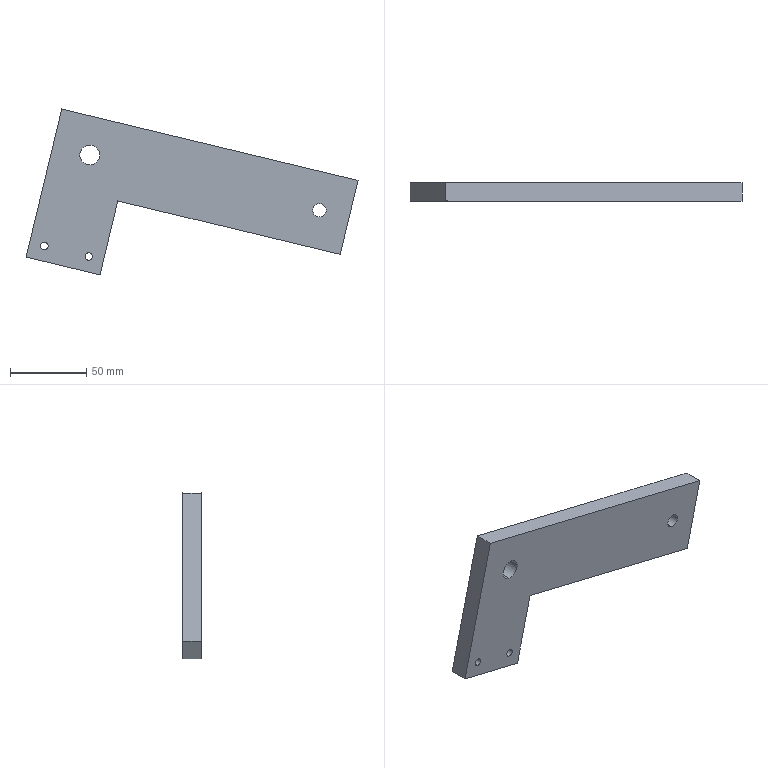Component | SolidWorks | SpringPullPlate-1 | 1 solid | 16 faces | box 217.86 x 12 x 108.93 mm | volume 147206 mm3 | cylinder 8 | plane 8 | commonest cylinder face diameters 5 x4 8.8 x2 13 x2
build123d program:
from build123d import *

# Parameters (mm, degrees)
SKETCH1_R                   = 6.5
EXTRUDE1_DEPTH              = 12
M10X1_25_TAPPED_HOLE1_D     = 8.8
M10X1_25_TAPPED_HOLE1_DEPTH = 26.25
M10X1_25_TAPPED_HOLE1_TIP   = 2.644
M6_TAPPED_HOLE1_D           = 5
M6_TAPPED_HOLE1_DEPTH       = 17
M6_TAPPED_HOLE1_TIP         = 1.502


with BuildPart() as part:
    # Sketch1 → Extrude1 (new body)
    with BuildSketch(Plane.XY):
        Polygon((-30.524, 33.502), (-30.524, -166.498), (69.476, -166.498), (69.476, -116.498), (19.476, -116.498), (19.476, 33.502), align=None)
        with Locations((-5.524, -141.498)):
            Circle(SKETCH1_R, mode=Mode.SUBTRACT)
    extrude(amount=EXTRUDE1_DEPTH)

    # M10x1.25 Tapped Hole1
    with Locations(Plane(origin=(-5.524, 13.502, 12), x_dir=(1, 0, 0), z_dir=(0, 0, 1))):
        with Locations((0, 0)):
            Hole(M10X1_25_TAPPED_HOLE1_D / 2, depth=M10X1_25_TAPPED_HOLE1_DEPTH)
            with Locations((0, 0, -(M10X1_25_TAPPED_HOLE1_DEPTH + M10X1_25_TAPPED_HOLE1_TIP / 2))):  # 118° drill point
                Cone(0, M10X1_25_TAPPED_HOLE1_D / 2, M10X1_25_TAPPED_HOLE1_TIP, mode=Mode.SUBTRACT)

    # M6 Tapped Hole1
    with Locations(Plane(origin=(59.476, -126.498, 12), x_dir=(1, 0, 0), z_dir=(0, 0, 1))):
        with Locations((0, 0), (0, -30)):
            Hole(M6_TAPPED_HOLE1_D / 2, depth=M6_TAPPED_HOLE1_DEPTH)
            with Locations((0, 0, -(M6_TAPPED_HOLE1_DEPTH + M6_TAPPED_HOLE1_TIP / 2))):  # 118° drill point
                Cone(0, M6_TAPPED_HOLE1_D / 2, M6_TAPPED_HOLE1_TIP, mode=Mode.SUBTRACT)


solid = part.part

# Placed as in the assembly
solid = solid.moved(Location((386.487, 406.983, -247.005), (90, 0, -103.543)))
STEP:
#1=CARTESIAN_POINT('',(9.849,16.023,-10.739));
#2=VERTEX_POINT('',#1);
#3=CARTESIAN_POINT('',(9.803,16.023,-10.931));
#4=VERTEX_POINT('',#3);
#5=CARTESIAN_POINT('',(9.826,16.023,-10.835));
#6=DIRECTION('',(-0.,-1.,0.));
#7=DIRECTION('',(-0.2342,0.,-0.9722));
#8=AXIS2_PLACEMENT_3D('',#5,#6,#7);
#9=CIRCLE('',#8,0.09843);
#10=EDGE_CURVE('',#2,#4,#9,.T.);
#11=ORIENTED_EDGE('',*,*,#10,.F.);
#12=CARTESIAN_POINT('',(9.849,15.551,-10.739));
#13=VERTEX_POINT('',#12);
#14=CARTESIAN_POINT('',(9.849,15.551,-10.739));
#15=DIRECTION('',(-0.,-1.,0.));
#16=VECTOR('',#15,39.37);
#17=LINE('',#14,#16);
#18=EDGE_CURVE('',#2,#13,#17,.T.);
#19=ORIENTED_EDGE('',*,*,#18,.T.);
#20=CARTESIAN_POINT('',(9.803,15.551,-10.931));
#21=VERTEX_POINT('',#20);
#22=CARTESIAN_POINT('',(9.826,15.551,-10.835));
#23=DIRECTION('',(-0.,-1.,0.));
#24=DIRECTION('',(-0.2342,0.,-0.9722));
#25=AXIS2_PLACEMENT_3D('',#22,#23,#24);
#26=CIRCLE('',#25,0.09843);
#27=EDGE_CURVE('',#13,#21,#26,.T.);
#28=ORIENTED_EDGE('',*,*,#27,.T.);
#29=CARTESIAN_POINT('',(9.803,15.551,-10.931));
#30=DIRECTION('',(-0.,-1.,0.));
#31=VECTOR('',#30,39.37);
#32=LINE('',#29,#31);
#33=EDGE_CURVE('',#4,#21,#32,.T.);
#34=ORIENTED_EDGE('',*,*,#33,.F.);
#35=EDGE_LOOP('',(#11,#19,#28,#34));
#36=FACE_OUTER_BOUND('',#35,.T.);
#37=CARTESIAN_POINT('',(9.826,15.551,-10.835));
#38=DIRECTION('',(-0.,-1.,0.));
#39=DIRECTION('',(-0.2342,0.,-0.9722));
#40=AXIS2_PLACEMENT_3D('',#37,#38,#39);
#41=CYLINDRICAL_SURFACE('',#40,0.09843);
#42=ADVANCED_FACE('',(#36),#41,.F.);
#43=CARTESIAN_POINT('',(8.701,16.023,-10.463));
#44=VERTEX_POINT('',#43);
#45=CARTESIAN_POINT('',(8.655,16.023,-10.654));
#46=VERTEX_POINT('',#45);
#47=CARTESIAN_POINT('',(8.678,16.023,-10.558));
#48=DIRECTION('',(-0.,-1.,0.));
#49=DIRECTION('',(-0.2342,0.,-0.9722));
#50=AXIS2_PLACEMENT_3D('',#47,#48,#49);
#51=CIRCLE('',#50,0.09843);
#52=EDGE_CURVE('',#44,#46,#51,.T.);
#53=ORIENTED_EDGE('',*,*,#52,.F.);
#54=CARTESIAN_POINT('',(8.701,15.551,-10.463));
#55=VERTEX_POINT('',#54);
#56=CARTESIAN_POINT('',(8.701,15.551,-10.463));
#57=DIRECTION('',(-0.,-1.,0.));
#58=VECTOR('',#57,39.37);
#59=LINE('',#56,#58);
#60=EDGE_CURVE('',#44,#55,#59,.T.);
#61=ORIENTED_EDGE('',*,*,#60,.T.);
#62=CARTESIAN_POINT('',(8.655,15.551,-10.654));
#63=VERTEX_POINT('',#62);
#64=CARTESIAN_POINT('',(8.678,15.551,-10.558));
#65=DIRECTION('',(-0.,-1.,0.));
#66=DIRECTION('',(-0.2342,0.,-0.9722));
#67=AXIS2_PLACEMENT_3D('',#64,#65,#66);
#68=CIRCLE('',#67,0.09843);
#69=EDGE_CURVE('',#55,#63,#68,.T.);
#70=ORIENTED_EDGE('',*,*,#69,.T.);
#71=CARTESIAN_POINT('',(8.655,15.551,-10.654));
#72=DIRECTION('',(-0.,-1.,0.));
#73=VECTOR('',#72,39.37);
#74=LINE('',#71,#73);
#75=EDGE_CURVE('',#46,#63,#74,.T.);
#76=ORIENTED_EDGE('',*,*,#75,.F.);
#77=EDGE_LOOP('',(#53,#61,#70,#76));
#78=FACE_OUTER_BOUND('',#77,.T.);
#79=CARTESIAN_POINT('',(8.678,15.551,-10.558));
#80=DIRECTION('',(-0.,-1.,0.));
#81=DIRECTION('',(-0.2342,0.,-0.9722));
#82=AXIS2_PLACEMENT_3D('',#79,#80,#81);
#83=CYLINDRICAL_SURFACE('',#82,0.09843);
#84=ADVANCED_FACE('',(#78),#83,.F.);
#85=CARTESIAN_POINT('',(15.824,16.023,-9.469));
#86=VERTEX_POINT('',#85);
#87=CARTESIAN_POINT('',(15.743,16.023,-9.806));
#88=VERTEX_POINT('',#87);
#89=CARTESIAN_POINT('',(15.784,16.023,-9.638));
#90=DIRECTION('',(-0.,-1.,0.));
#91=DIRECTION('',(-0.2342,0.,-0.9722));
#92=AXIS2_PLACEMENT_3D('',#89,#90,#91);
#93=CIRCLE('',#92,0.1732);
#94=EDGE_CURVE('',#86,#88,#93,.T.);
#95=ORIENTED_EDGE('',*,*,#94,.F.);
#96=CARTESIAN_POINT('',(15.824,15.551,-9.469));
#97=VERTEX_POINT('',#96);
#98=CARTESIAN_POINT('',(15.824,15.551,-9.469));
#99=DIRECTION('',(-0.,-1.,0.));
#100=VECTOR('',#99,39.37);
#101=LINE('',#98,#100);
#102=EDGE_CURVE('',#86,#97,#101,.T.);
#103=ORIENTED_EDGE('',*,*,#102,.T.);
#104=CARTESIAN_POINT('',(15.743,15.551,-9.806));
#105=VERTEX_POINT('',#104);
#106=CARTESIAN_POINT('',(15.784,15.551,-9.638));
#107=DIRECTION('',(-0.,-1.,0.));
#108=DIRECTION('',(-0.2342,0.,-0.9722));
#109=AXIS2_PLACEMENT_3D('',#106,#107,#108);
#110=CIRCLE('',#109,0.1732);
#111=EDGE_CURVE('',#97,#105,#110,.T.);
#112=ORIENTED_EDGE('',*,*,#111,.T.);
#113=CARTESIAN_POINT('',(15.743,15.551,-9.806));
#114=DIRECTION('',(-0.,-1.,0.));
#115=VECTOR('',#114,39.37);
#116=LINE('',#113,#115);
#117=EDGE_CURVE('',#88,#105,#116,.T.);
#118=ORIENTED_EDGE('',*,*,#117,.F.);
#119=EDGE_LOOP('',(#95,#103,#112,#118));
#120=FACE_OUTER_BOUND('',#119,.T.);
#121=CARTESIAN_POINT('',(15.784,15.551,-9.638));
#122=DIRECTION('',(-0.,-1.,0.));
#123=DIRECTION('',(-0.2342,0.,-0.9722));
#124=AXIS2_PLACEMENT_3D('',#121,#122,#123);
#125=CYLINDRICAL_SURFACE('',#124,0.1732);
#126=ADVANCED_FACE('',(#120),#125,.F.);
#127=CARTESIAN_POINT('',(9.911,15.551,-7.96));
#128=VERTEX_POINT('',#127);
#129=CARTESIAN_POINT('',(9.791,15.551,-8.457));
#130=VERTEX_POINT('',#129);
#131=CARTESIAN_POINT('',(9.851,15.551,-8.209));
#132=DIRECTION('',(-0.,-1.,0.));
#133=DIRECTION('',(-0.2342,0.,-0.9722));
#134=AXIS2_PLACEMENT_3D('',#131,#132,#133);
#135=CIRCLE('',#134,0.2559);
#136=EDGE_CURVE('',#128,#130,#135,.T.);
#137=ORIENTED_EDGE('',*,*,#136,.T.);
#138=CARTESIAN_POINT('',(9.791,16.023,-8.457));
#139=VERTEX_POINT('',#138);
#140=CARTESIAN_POINT('',(9.791,15.551,-8.457));
#141=DIRECTION('',(0.,1.,-0.));
#142=VECTOR('',#141,39.37);
#143=LINE('',#140,#142);
#144=EDGE_CURVE('',#130,#139,#143,.T.);
#145=ORIENTED_EDGE('',*,*,#144,.T.);
#146=CARTESIAN_POINT('',(9.911,16.023,-7.96));
#147=VERTEX_POINT('',#146);
#148=CARTESIAN_POINT('',(9.851,16.023,-8.209));
#149=DIRECTION('',(-0.,-1.,0.));
#150=DIRECTION('',(-0.2342,0.,-0.9722));
#151=AXIS2_PLACEMENT_3D('',#148,#149,#150);
#152=CIRCLE('',#151,0.2559);
#153=EDGE_CURVE('',#147,#139,#152,.T.);
#154=ORIENTED_EDGE('',*,*,#153,.F.);
#155=CARTESIAN_POINT('',(9.911,15.551,-7.96));
#156=DIRECTION('',(0.,1.,-0.));
#157=VECTOR('',#156,39.37);
#158=LINE('',#155,#157);
#159=EDGE_CURVE('',#128,#147,#158,.T.);
#160=ORIENTED_EDGE('',*,*,#159,.F.);
#161=EDGE_LOOP('',(#137,#145,#154,#160));
#162=FACE_OUTER_BOUND('',#161,.T.);
#163=CARTESIAN_POINT('',(9.851,15.551,-8.209));
#164=DIRECTION('',(0.,1.,-0.));
#165=DIRECTION('',(0.2342,0.,0.9722));
#166=AXIS2_PLACEMENT_3D('',#163,#164,#165);
#167=CYLINDRICAL_SURFACE('',#166,0.2559);
#168=ADVANCED_FACE('',(#162),#167,.F.);
#169=CARTESIAN_POINT('',(9.826,15.551,-10.835));
#170=DIRECTION('',(-0.,-1.,0.));
#171=DIRECTION('',(-0.2342,0.,-0.9722));
#172=AXIS2_PLACEMENT_3D('',#169,#170,#171);
#173=CIRCLE('',#172,0.09843);
#174=EDGE_CURVE('',#21,#13,#173,.T.);
#175=ORIENTED_EDGE('',*,*,#174,.F.);
#176=ORIENTED_EDGE('',*,*,#27,.F.);
#177=EDGE_LOOP('',(#175,#176));
#178=FACE_BOUND('',#177,.T.);
#179=CARTESIAN_POINT('',(8.678,15.551,-10.558));
#180=DIRECTION('',(-0.,-1.,0.));
#181=DIRECTION('',(-0.2342,0.,-0.9722));
#182=AXIS2_PLACEMENT_3D('',#179,#180,#181);
#183=CIRCLE('',#182,0.09843);
#184=EDGE_CURVE('',#63,#55,#183,.T.);
#185=ORIENTED_EDGE('',*,*,#184,.F.);
#186=ORIENTED_EDGE('',*,*,#69,.F.);
#187=EDGE_LOOP('',(#185,#186));
#188=FACE_BOUND('',#187,.T.);
#189=CARTESIAN_POINT('',(15.784,15.551,-9.638));
#190=DIRECTION('',(-0.,-1.,0.));
#191=DIRECTION('',(-0.2342,0.,-0.9722));
#192=AXIS2_PLACEMENT_3D('',#189,#190,#191);
#193=CIRCLE('',#192,0.1732);
#194=EDGE_CURVE('',#105,#97,#193,.T.);
#195=ORIENTED_EDGE('',*,*,#194,.F.);
#196=ORIENTED_EDGE('',*,*,#111,.F.);
#197=EDGE_LOOP('',(#195,#196));
#198=FACE_BOUND('',#197,.T.);
#199=CARTESIAN_POINT('',(9.125,15.551,-7.021));
#200=VERTEX_POINT('',#199);
#201=CARTESIAN_POINT('',(8.203,15.551,-10.849));
#202=VERTEX_POINT('',#201);
#203=CARTESIAN_POINT('',(9.125,15.551,-7.021));
#204=DIRECTION('',(-0.2342,-0.,-0.9722));
#205=VECTOR('',#204,39.37);
#206=LINE('',#203,#205);
#207=EDGE_CURVE('',#200,#202,#206,.T.);
#208=ORIENTED_EDGE('',*,*,#207,.T.);
#209=CARTESIAN_POINT('',(10.116,15.551,-11.31));
#210=VERTEX_POINT('',#209);
#211=CARTESIAN_POINT('',(8.203,15.551,-10.849));
#212=DIRECTION('',(0.9722,-0.,-0.2342));
#213=VECTOR('',#212,39.37);
#214=LINE('',#211,#213);
#215=EDGE_CURVE('',#202,#210,#214,.T.);
#216=ORIENTED_EDGE('',*,*,#215,.T.);
#217=CARTESIAN_POINT('',(10.577,15.551,-9.396));
#218=VERTEX_POINT('',#217);
#219=CARTESIAN_POINT('',(10.116,15.551,-11.31));
#220=DIRECTION('',(0.2342,0.,0.9722));
#221=VECTOR('',#220,39.37);
#222=LINE('',#219,#221);
#223=EDGE_CURVE('',#210,#218,#222,.T.);
#224=ORIENTED_EDGE('',*,*,#223,.T.);
#225=CARTESIAN_POINT('',(16.319,15.551,-10.779));
#226=VERTEX_POINT('',#225);
#227=CARTESIAN_POINT('',(10.577,15.551,-9.396));
#228=DIRECTION('',(0.9722,-0.,-0.2342));
#229=VECTOR('',#228,39.37);
#230=LINE('',#227,#229);
#231=EDGE_CURVE('',#218,#226,#230,.T.);
#232=ORIENTED_EDGE('',*,*,#231,.T.);
#233=CARTESIAN_POINT('',(16.78,15.551,-8.865));
#234=VERTEX_POINT('',#233);
#235=CARTESIAN_POINT('',(16.319,15.551,-10.779));
#236=DIRECTION('',(0.2342,0.,0.9722));
#237=VECTOR('',#236,39.37);
#238=LINE('',#235,#237);
#239=EDGE_CURVE('',#226,#234,#238,.T.);
#240=ORIENTED_EDGE('',*,*,#239,.T.);
#241=CARTESIAN_POINT('',(16.78,15.551,-8.865));
#242=DIRECTION('',(-0.9722,0.,0.2342));
#243=VECTOR('',#242,39.37);
#244=LINE('',#241,#243);
#245=EDGE_CURVE('',#234,#200,#244,.T.);
#246=ORIENTED_EDGE('',*,*,#245,.T.);
#247=EDGE_LOOP('',(#208,#216,#224,#232,#240,#246));
#248=FACE_OUTER_BOUND('',#247,.T.);
#249=ORIENTED_EDGE('',*,*,#136,.F.);
#250=CARTESIAN_POINT('',(9.851,15.551,-8.209));
#251=DIRECTION('',(-0.,-1.,0.));
#252=DIRECTION('',(-0.2342,0.,-0.9722));
#253=AXIS2_PLACEMENT_3D('',#250,#251,#252);
#254=CIRCLE('',#253,0.2559);
#255=EDGE_CURVE('',#130,#128,#254,.T.);
#256=ORIENTED_EDGE('',*,*,#255,.F.);
#257=EDGE_LOOP('',(#249,#256));
#258=FACE_BOUND('',#257,.T.);
#259=CARTESIAN_POINT('',(8.203,15.551,-10.849));
#260=DIRECTION('',(-0.,-1.,0.));
#261=DIRECTION('',(-0.2342,-0.,-0.9722));
#262=AXIS2_PLACEMENT_3D('',#259,#260,#261);
#263=PLANE('',#262);
#264=ADVANCED_FACE('',(#178,#188,#198,#248,#258),#263,.T.);
#265=CARTESIAN_POINT('',(9.826,16.023,-10.835));
#266=DIRECTION('',(-0.,-1.,0.));
#267=DIRECTION('',(-0.2342,0.,-0.9722));
#268=AXIS2_PLACEMENT_3D('',#265,#266,#267);
#269=CIRCLE('',#268,0.09843);
#270=EDGE_CURVE('',#4,#2,#269,.T.);
#271=ORIENTED_EDGE('',*,*,#270,.T.);
#272=ORIENTED_EDGE('',*,*,#10,.T.);
#273=EDGE_LOOP('',(#271,#272));
#274=FACE_BOUND('',#273,.T.);
#275=CARTESIAN_POINT('',(8.678,16.023,-10.558));
#276=DIRECTION('',(-0.,-1.,0.));
#277=DIRECTION('',(-0.2342,0.,-0.9722));
#278=AXIS2_PLACEMENT_3D('',#275,#276,#277);
#279=CIRCLE('',#278,0.09843);
#280=EDGE_CURVE('',#46,#44,#279,.T.);
#281=ORIENTED_EDGE('',*,*,#280,.T.);
#282=ORIENTED_EDGE('',*,*,#52,.T.);
#283=EDGE_LOOP('',(#281,#282));
#284=FACE_BOUND('',#283,.T.);
#285=CARTESIAN_POINT('',(15.784,16.023,-9.638));
#286=DIRECTION('',(-0.,-1.,0.));
#287=DIRECTION('',(-0.2342,0.,-0.9722));
#288=AXIS2_PLACEMENT_3D('',#285,#286,#287);
#289=CIRCLE('',#288,0.1732);
#290=EDGE_CURVE('',#88,#86,#289,.T.);
#291=ORIENTED_EDGE('',*,*,#290,.T.);
#292=ORIENTED_EDGE('',*,*,#94,.T.);
#293=EDGE_LOOP('',(#291,#292));
#294=FACE_BOUND('',#293,.T.);
#295=CARTESIAN_POINT('',(9.125,16.023,-7.021));
#296=VERTEX_POINT('',#295);
#297=CARTESIAN_POINT('',(8.203,16.023,-10.849));
#298=VERTEX_POINT('',#297);
#299=CARTESIAN_POINT('',(9.125,16.023,-7.021));
#300=DIRECTION('',(-0.2342,-0.,-0.9722));
#301=VECTOR('',#300,39.37);
#302=LINE('',#299,#301);
#303=EDGE_CURVE('',#296,#298,#302,.T.);
#304=ORIENTED_EDGE('',*,*,#303,.F.);
#305=CARTESIAN_POINT('',(16.78,16.023,-8.865));
#306=VERTEX_POINT('',#305);
#307=CARTESIAN_POINT('',(16.78,16.023,-8.865));
#308=DIRECTION('',(-0.9722,0.,0.2342));
#309=VECTOR('',#308,39.37);
#310=LINE('',#307,#309);
#311=EDGE_CURVE('',#306,#296,#310,.T.);
#312=ORIENTED_EDGE('',*,*,#311,.F.);
#313=CARTESIAN_POINT('',(16.319,16.023,-10.779));
#314=VERTEX_POINT('',#313);
#315=CARTESIAN_POINT('',(16.319,16.023,-10.779));
#316=DIRECTION('',(0.2342,0.,0.9722));
#317=VECTOR('',#316,39.37);
#318=LINE('',#315,#317);
#319=EDGE_CURVE('',#314,#306,#318,.T.);
#320=ORIENTED_EDGE('',*,*,#319,.F.);
#321=CARTESIAN_POINT('',(10.577,16.023,-9.396));
#322=VERTEX_POINT('',#321);
#323=CARTESIAN_POINT('',(10.577,16.023,-9.396));
#324=DIRECTION('',(0.9722,-0.,-0.2342));
#325=VECTOR('',#324,39.37);
#326=LINE('',#323,#325);
#327=EDGE_CURVE('',#322,#314,#326,.T.);
#328=ORIENTED_EDGE('',*,*,#327,.F.);
#329=CARTESIAN_POINT('',(10.116,16.023,-11.31));
#330=VERTEX_POINT('',#329);
#331=CARTESIAN_POINT('',(10.116,16.023,-11.31));
#332=DIRECTION('',(0.2342,0.,0.9722));
#333=VECTOR('',#332,39.37);
#334=LINE('',#331,#333);
#335=EDGE_CURVE('',#330,#322,#334,.T.);
#336=ORIENTED_EDGE('',*,*,#335,.F.);
#337=CARTESIAN_POINT('',(8.203,16.023,-10.849));
#338=DIRECTION('',(0.9722,-0.,-0.2342));
#339=VECTOR('',#338,39.37);
#340=LINE('',#337,#339);
#341=EDGE_CURVE('',#298,#330,#340,.T.);
#342=ORIENTED_EDGE('',*,*,#341,.F.);
#343=EDGE_LOOP('',(#304,#312,#320,#328,#336,#342));
#344=FACE_OUTER_BOUND('',#343,.T.);
#345=ORIENTED_EDGE('',*,*,#153,.T.);
#346=CARTESIAN_POINT('',(9.851,16.023,-8.209));
#347=DIRECTION('',(-0.,-1.,0.));
#348=DIRECTION('',(-0.2342,0.,-0.9722));
#349=AXIS2_PLACEMENT_3D('',#346,#347,#348);
#350=CIRCLE('',#349,0.2559);
#351=EDGE_CURVE('',#139,#147,#350,.T.);
#352=ORIENTED_EDGE('',*,*,#351,.T.);
#353=EDGE_LOOP('',(#345,#352));
#354=FACE_BOUND('',#353,.T.);
#355=CARTESIAN_POINT('',(8.203,16.023,-10.849));
#356=DIRECTION('',(-0.,-1.,0.));
#357=DIRECTION('',(-0.2342,-0.,-0.9722));
#358=AXIS2_PLACEMENT_3D('',#355,#356,#357);
#359=PLANE('',#358);
#360=ADVANCED_FACE('',(#274,#284,#294,#344,#354),#359,.F.);
#361=ORIENTED_EDGE('',*,*,#303,.T.);
#362=CARTESIAN_POINT('',(8.203,15.551,-10.849));
#363=DIRECTION('',(0.,1.,-0.));
#364=VECTOR('',#363,39.37);
#365=LINE('',#362,#364);
#366=EDGE_CURVE('',#202,#298,#365,.T.);
#367=ORIENTED_EDGE('',*,*,#366,.F.);
#368=ORIENTED_EDGE('',*,*,#207,.F.);
#369=CARTESIAN_POINT('',(9.125,15.551,-7.021));
#370=DIRECTION('',(0.,1.,-0.));
#371=VECTOR('',#370,39.37);
#372=LINE('',#369,#371);
#373=EDGE_CURVE('',#200,#296,#372,.T.);
#374=ORIENTED_EDGE('',*,*,#373,.T.);
#375=EDGE_LOOP('',(#361,#367,#368,#374));
#376=FACE_OUTER_BOUND('',#375,.T.);
#377=CARTESIAN_POINT('',(9.125,15.551,-7.021));
#378=DIRECTION('',(0.9722,-0.,-0.2342));
#379=DIRECTION('',(-0.,-1.,0.));
#380=AXIS2_PLACEMENT_3D('',#377,#378,#379);
#381=PLANE('',#380);
#382=ADVANCED_FACE('',(#376),#381,.F.);
#383=ORIENTED_EDGE('',*,*,#341,.T.);
#384=CARTESIAN_POINT('',(10.116,15.551,-11.31));
#385=DIRECTION('',(0.,1.,-0.));
#386=VECTOR('',#385,39.37);
#387=LINE('',#384,#386);
#388=EDGE_CURVE('',#210,#330,#387,.T.);
#389=ORIENTED_EDGE('',*,*,#388,.F.);
#390=ORIENTED_EDGE('',*,*,#215,.F.);
#391=ORIENTED_EDGE('',*,*,#366,.T.);
#392=EDGE_LOOP('',(#383,#389,#390,#391));
#393=FACE_OUTER_BOUND('',#392,.T.);
#394=CARTESIAN_POINT('',(8.203,15.551,-10.849));
#395=DIRECTION('',(0.2342,0.,0.9722));
#396=DIRECTION('',(-0.,-1.,0.));
#397=AXIS2_PLACEMENT_3D('',#394,#395,#396);
#398=PLANE('',#397);
#399=ADVANCED_FACE('',(#393),#398,.F.);
#400=ORIENTED_EDGE('',*,*,#335,.T.);
#401=CARTESIAN_POINT('',(10.577,15.551,-9.396));
#402=DIRECTION('',(0.,1.,-0.));
#403=VECTOR('',#402,39.37);
#404=LINE('',#401,#403);
#405=EDGE_CURVE('',#218,#322,#404,.T.);
#406=ORIENTED_EDGE('',*,*,#405,.F.);
#407=ORIENTED_EDGE('',*,*,#223,.F.);
#408=ORIENTED_EDGE('',*,*,#388,.T.);
#409=EDGE_LOOP('',(#400,#406,#407,#408));
#410=FACE_OUTER_BOUND('',#409,.T.);
#411=CARTESIAN_POINT('',(10.116,15.551,-11.31));
#412=DIRECTION('',(-0.9722,0.,0.2342));
#413=DIRECTION('',(-0.2342,-0.,-0.9722));
#414=AXIS2_PLACEMENT_3D('',#411,#412,#413);
#415=PLANE('',#414);
#416=ADVANCED_FACE('',(#410),#415,.F.);
#417=ORIENTED_EDGE('',*,*,#327,.T.);
#418=CARTESIAN_POINT('',(16.319,15.551,-10.779));
#419=DIRECTION('',(0.,1.,-0.));
#420=VECTOR('',#419,39.37);
#421=LINE('',#418,#420);
#422=EDGE_CURVE('',#226,#314,#421,.T.);
#423=ORIENTED_EDGE('',*,*,#422,.F.);
#424=ORIENTED_EDGE('',*,*,#231,.F.);
#425=ORIENTED_EDGE('',*,*,#405,.T.);
#426=EDGE_LOOP('',(#417,#423,#424,#425));
#427=FACE_OUTER_BOUND('',#426,.T.);
#428=CARTESIAN_POINT('',(10.577,15.551,-9.396));
#429=DIRECTION('',(0.2342,0.,0.9722));
#430=DIRECTION('',(-0.,-1.,0.));
#431=AXIS2_PLACEMENT_3D('',#428,#429,#430);
#432=PLANE('',#431);
#433=ADVANCED_FACE('',(#427),#432,.F.);
#434=ORIENTED_EDGE('',*,*,#319,.T.);
#435=CARTESIAN_POINT('',(16.78,15.551,-8.865));
#436=DIRECTION('',(0.,1.,-0.));
#437=VECTOR('',#436,39.37);
#438=LINE('',#435,#437);
#439=EDGE_CURVE('',#234,#306,#438,.T.);
#440=ORIENTED_EDGE('',*,*,#439,.F.);
#441=ORIENTED_EDGE('',*,*,#239,.F.);
#442=ORIENTED_EDGE('',*,*,#422,.T.);
#443=EDGE_LOOP('',(#434,#440,#441,#442));
#444=FACE_OUTER_BOUND('',#443,.T.);
#445=CARTESIAN_POINT('',(16.319,15.551,-10.779));
#446=DIRECTION('',(-0.9722,0.,0.2342));
#447=DIRECTION('',(-0.2342,-0.,-0.9722));
#448=AXIS2_PLACEMENT_3D('',#445,#446,#447);
#449=PLANE('',#448);
#450=ADVANCED_FACE('',(#444),#449,.F.);
#451=ORIENTED_EDGE('',*,*,#311,.T.);
#452=ORIENTED_EDGE('',*,*,#373,.F.);
#453=ORIENTED_EDGE('',*,*,#245,.F.);
#454=ORIENTED_EDGE('',*,*,#439,.T.);
#455=EDGE_LOOP('',(#451,#452,#453,#454));
#456=FACE_OUTER_BOUND('',#455,.T.);
#457=CARTESIAN_POINT('',(16.78,15.551,-8.865));
#458=DIRECTION('',(-0.2342,-0.,-0.9722));
#459=DIRECTION('',(0.9722,-0.,-0.2342));
#460=AXIS2_PLACEMENT_3D('',#457,#458,#459);
#461=PLANE('',#460);
#462=ADVANCED_FACE('',(#456),#461,.F.);
#463=ORIENTED_EDGE('',*,*,#144,.F.);
#464=ORIENTED_EDGE('',*,*,#255,.T.);
#465=ORIENTED_EDGE('',*,*,#159,.T.);
#466=ORIENTED_EDGE('',*,*,#351,.F.);
#467=EDGE_LOOP('',(#463,#464,#465,#466));
#468=FACE_OUTER_BOUND('',#467,.T.);
#469=CARTESIAN_POINT('',(9.851,15.551,-8.209));
#470=DIRECTION('',(0.,1.,-0.));
#471=DIRECTION('',(0.2342,0.,0.9722));
#472=AXIS2_PLACEMENT_3D('',#469,#470,#471);
#473=CYLINDRICAL_SURFACE('',#472,0.2559);
#474=ADVANCED_FACE('',(#468),#473,.F.);
#475=ORIENTED_EDGE('',*,*,#102,.F.);
#476=ORIENTED_EDGE('',*,*,#290,.F.);
#477=ORIENTED_EDGE('',*,*,#117,.T.);
#478=ORIENTED_EDGE('',*,*,#194,.T.);
#479=EDGE_LOOP('',(#475,#476,#477,#478));
#480=FACE_OUTER_BOUND('',#479,.T.);
#481=CARTESIAN_POINT('',(15.784,15.551,-9.638));
#482=DIRECTION('',(-0.,-1.,0.));
#483=DIRECTION('',(-0.2342,0.,-0.9722));
#484=AXIS2_PLACEMENT_3D('',#481,#482,#483);
#485=CYLINDRICAL_SURFACE('',#484,0.1732);
#486=ADVANCED_FACE('',(#480),#485,.F.);
#487=ORIENTED_EDGE('',*,*,#60,.F.);
#488=ORIENTED_EDGE('',*,*,#280,.F.);
#489=ORIENTED_EDGE('',*,*,#75,.T.);
#490=ORIENTED_EDGE('',*,*,#184,.T.);
#491=EDGE_LOOP('',(#487,#488,#489,#490));
#492=FACE_OUTER_BOUND('',#491,.T.);
#493=CARTESIAN_POINT('',(8.678,15.551,-10.558));
#494=DIRECTION('',(-0.,-1.,0.));
#495=DIRECTION('',(-0.2342,0.,-0.9722));
#496=AXIS2_PLACEMENT_3D('',#493,#494,#495);
#497=CYLINDRICAL_SURFACE('',#496,0.09843);
#498=ADVANCED_FACE('',(#492),#497,.F.);
#499=ORIENTED_EDGE('',*,*,#18,.F.);
#500=ORIENTED_EDGE('',*,*,#270,.F.);
#501=ORIENTED_EDGE('',*,*,#33,.T.);
#502=ORIENTED_EDGE('',*,*,#174,.T.);
#503=EDGE_LOOP('',(#499,#500,#501,#502));
#504=FACE_OUTER_BOUND('',#503,.T.);
#505=CARTESIAN_POINT('',(9.826,15.551,-10.835));
#506=DIRECTION('',(-0.,-1.,0.));
#507=DIRECTION('',(-0.2342,0.,-0.9722));
#508=AXIS2_PLACEMENT_3D('',#505,#506,#507);
#509=CYLINDRICAL_SURFACE('',#508,0.09843);
#510=ADVANCED_FACE('',(#504),#509,.F.);
#511=CLOSED_SHELL('',(#42,#84,#126,#168,#264,#360,#382,#399,#416,#433,#450,#462,#474,#486,#498,#510));
#512=MANIFOLD_SOLID_BREP('',#511);
#513=CARTESIAN_POINT('',(0.,0.,0.));
#514=DIRECTION('',(0.,0.,1.));
#515=DIRECTION('',(1.,0.,0.));
#516=AXIS2_PLACEMENT_3D('',#513,#514,#515);
#517=(LENGTH_UNIT()NAMED_UNIT(*)SI_UNIT($,.METRE.));
#518=LENGTH_MEASURE_WITH_UNIT(LENGTH_MEASURE(0.0254),#517);
#519=DIMENSIONAL_EXPONENTS(1.,0.,0.,0.,0.,0.,0.);
#520=(CONVERSION_BASED_UNIT('',#518)LENGTH_UNIT()NAMED_UNIT(#519));
#521=UNCERTAINTY_MEASURE_WITH_UNIT(LENGTH_MEASURE(0.00001),#520,'','');
#522=(NAMED_UNIT(*)PLANE_ANGLE_UNIT()SI_UNIT($,.RADIAN.));
#523=(NAMED_UNIT(*)SI_UNIT($,.STERADIAN.)SOLID_ANGLE_UNIT());
#524=(GEOMETRIC_REPRESENTATION_CONTEXT(3)GLOBAL_UNCERTAINTY_ASSIGNED_CONTEXT((#521))GLOBAL_UNIT_ASSIGNED_CONTEXT((#520,#522,#523))REPRESENTATION_CONTEXT('',''));
#525=ADVANCED_BREP_SHAPE_REPRESENTATION('',(#512,#516),#524);
#526=COLOUR_RGB('',0.7922,0.8196,0.9333);
#527=FILL_AREA_STYLE_COLOUR('',#526);
#528=FILL_AREA_STYLE('',(#527));
#529=SURFACE_STYLE_FILL_AREA(#528);
#530=SURFACE_SIDE_STYLE('',(#529));
#531=SURFACE_STYLE_USAGE(.BOTH.,#530);
#532=PRESENTATION_STYLE_ASSIGNMENT((#531));
#533=STYLED_ITEM('',(#532),#512);
#534=PRESENTATION_LAYER_ASSIGNMENT('','',(#533));
#535=(LENGTH_UNIT()NAMED_UNIT(*)SI_UNIT($,.METRE.));
#536=LENGTH_MEASURE_WITH_UNIT(LENGTH_MEASURE(0.0254),#535);
#537=DIMENSIONAL_EXPONENTS(1.,0.,0.,0.,0.,0.,0.);
#538=(CONVERSION_BASED_UNIT('',#536)LENGTH_UNIT()NAMED_UNIT(#537));
#539=UNCERTAINTY_MEASURE_WITH_UNIT(LENGTH_MEASURE(0.00001),#538,'','');
#540=(NAMED_UNIT(*)PLANE_ANGLE_UNIT()SI_UNIT($,.RADIAN.));
#541=(NAMED_UNIT(*)SI_UNIT($,.STERADIAN.)SOLID_ANGLE_UNIT());
#542=(GEOMETRIC_REPRESENTATION_CONTEXT(3)GLOBAL_UNCERTAINTY_ASSIGNED_CONTEXT((#539))GLOBAL_UNIT_ASSIGNED_CONTEXT((#538,#540,#541))REPRESENTATION_CONTEXT('',''));
#543=MECHANICAL_DESIGN_GEOMETRIC_PRESENTATION_REPRESENTATION('',(#533),#542);